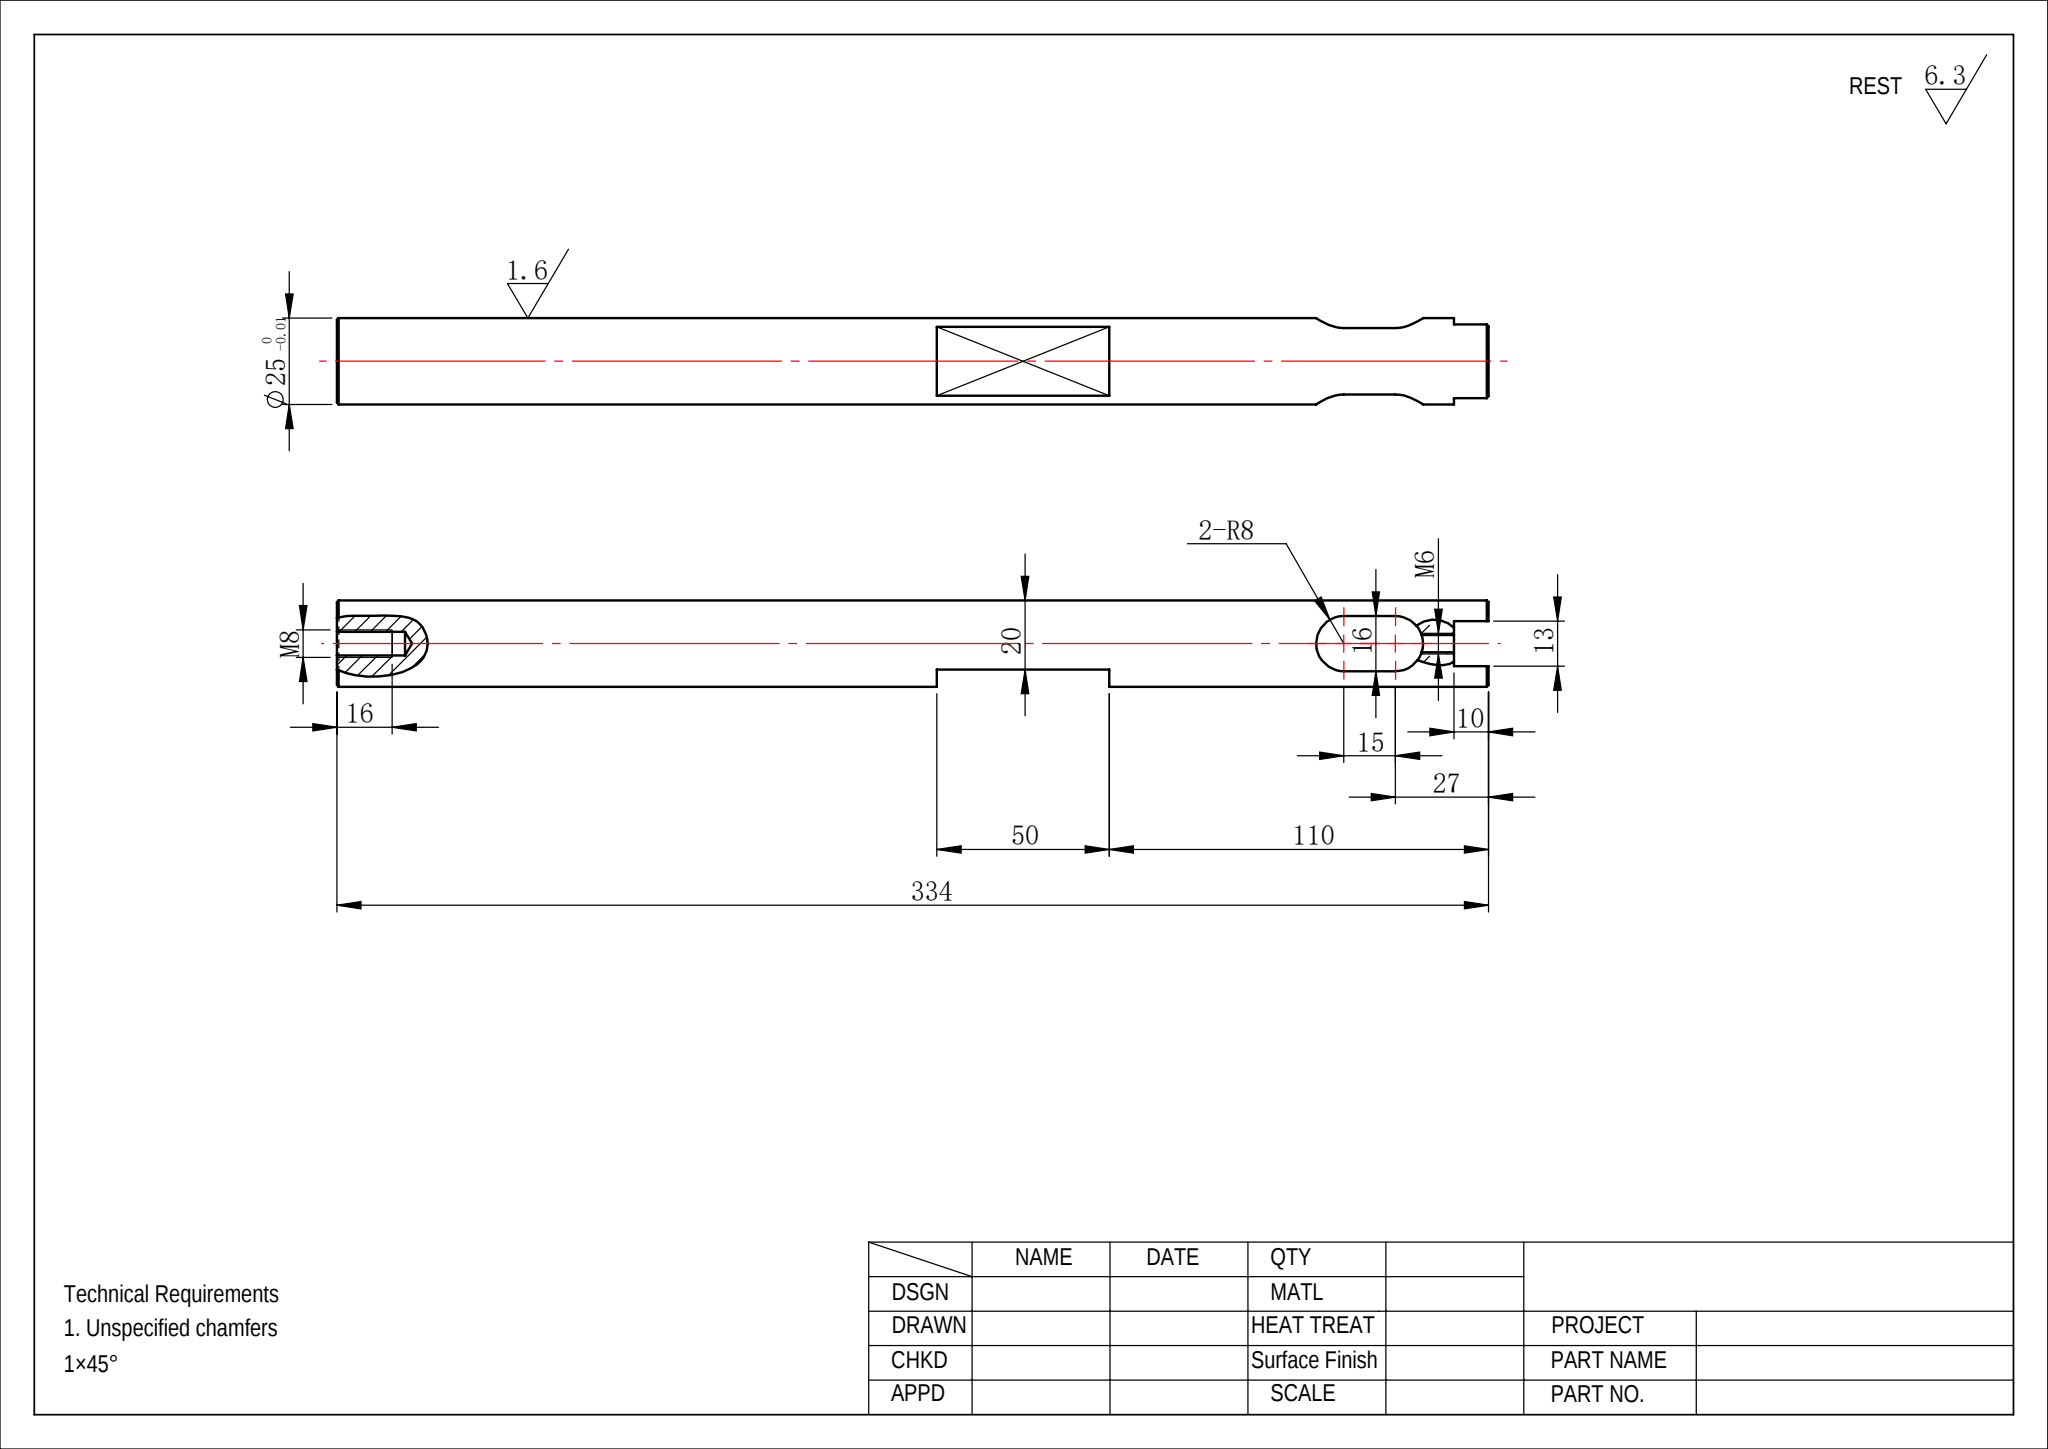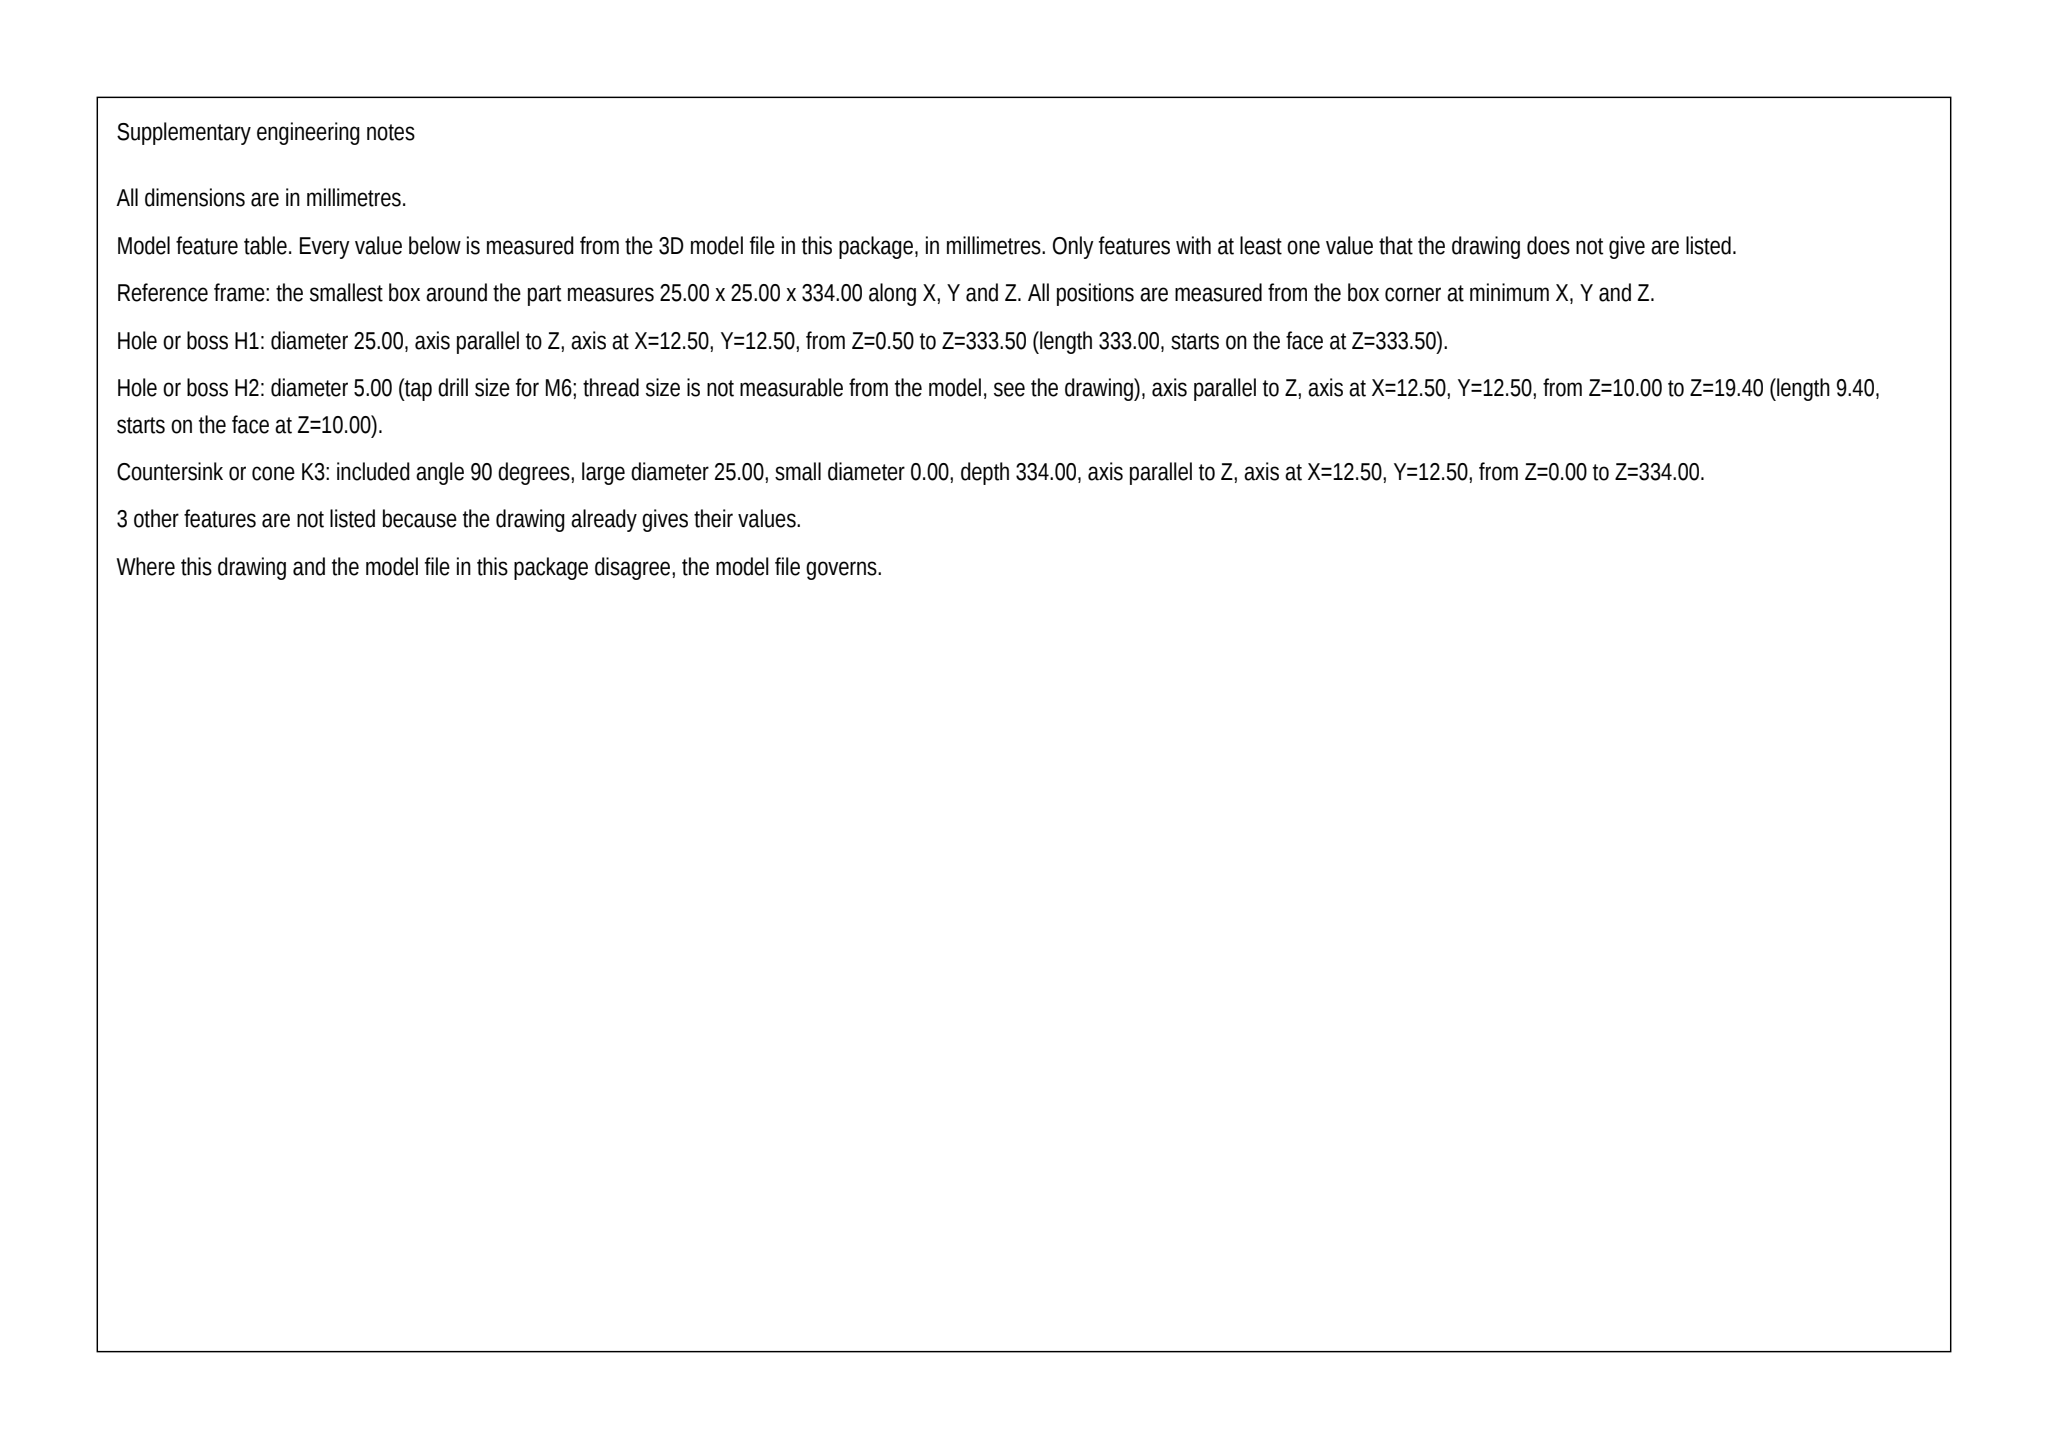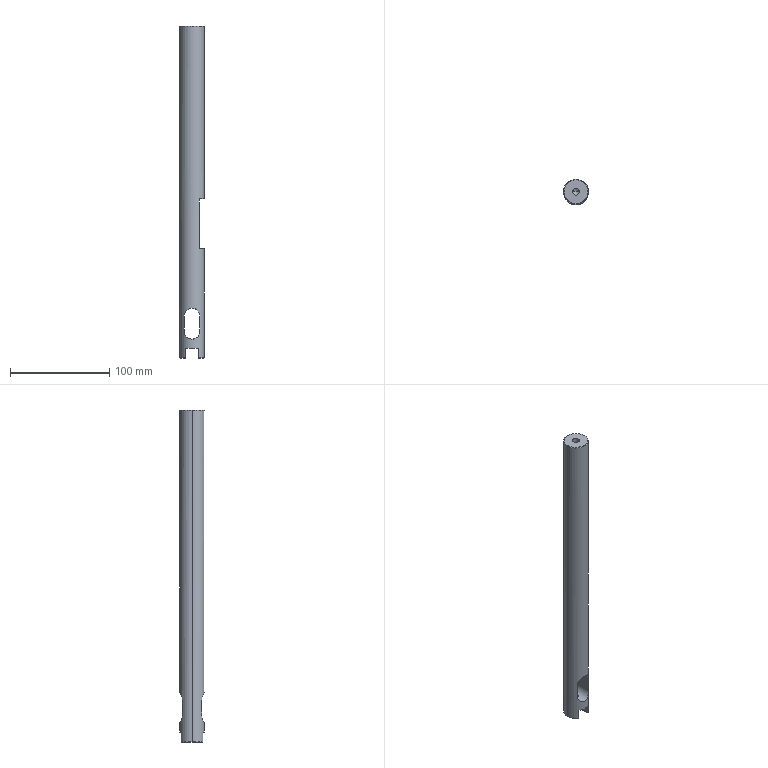Part | SolidWorks | mm | 1 solid | 27 faces | box 25 x 25 x 334 mm | volume 146109 mm3 | plane 11 | cylinder 9 | cone 7 | commonest cylinder face diameters 16 x3 5 x2 6.8 x2 25 x2
build123d program:
from build123d import *

# Parameters (mm, degrees)
SKETCH1_R             = 12.5
EXTRUDE1_DEPTH        = 334
SKETCH2_W             = 13
SKETCH2_H             = 26.185
CUT_EXTRUDE1_DEPTH    = 10
M8_TAPPED_HOLE1_D     = 6.8
M8_TAPPED_HOLE1_DEPTH = 19.75
M8_TAPPED_HOLE1_TIP   = 2.043
CUT_EXTRUDE3_DEPTH    = 25
SKETCH12_W            = 12.5
SKETCH12_H            = 10
SKETCH13_W            = 50
SKETCH13_H            = 120.795
CUT_EXTRUDE4_DEPTH    = 5
CHAMFER1_SIZE         = 0.5
M6_TAPPED_HOLE1_D     = 5
M6_TAPPED_HOLE1_DEPTH = 17
M6_TAPPED_HOLE1_TIP   = 1.502
SKETCH15_W            = 23.242
SKETCH15_H            = 67.222


with BuildPart() as part:
    # Sketch1 → Extrude1 (new body)
    with BuildSketch(Plane.XY):
        with Locations(Location((0, 0, 0), (0, 0, 180))):
            Circle(SKETCH1_R)
    extrude(amount=EXTRUDE1_DEPTH)

    # Sketch2 → Cut-Extrude1 (cut)
    with BuildSketch(Plane(origin=(0, 0, 0), x_dir=(-1, 0, 0), z_dir=(0, 0, -1))):
        with Locations((0, 0.2525)):
            Rectangle(SKETCH2_W, SKETCH2_H)
    extrude(amount=-CUT_EXTRUDE1_DEPTH, mode=Mode.SUBTRACT)

    # M8 Tapped Hole1
    with Locations(Plane.XY.offset(334)):
        with Locations((0, 0)):
            Hole(M8_TAPPED_HOLE1_D / 2, depth=M8_TAPPED_HOLE1_DEPTH)
            with Locations((0, 0, -(M8_TAPPED_HOLE1_DEPTH + M8_TAPPED_HOLE1_TIP / 2))):  # 118° drill point
                Cone(0, M8_TAPPED_HOLE1_D / 2, M8_TAPPED_HOLE1_TIP, mode=Mode.SUBTRACT)

    # Sketch7 → Cut-Extrude3 (cut, symmetric)
    with BuildSketch(Plane(origin=(0, 0, 0), x_dir=(1, 0, 0), z_dir=(0, 1, 0))):
        with BuildLine():
            Line((-8, -27), (-8, -42))
            ThreePointArc((-8, -42), (0, -50), (8, -42))
            Line((8, -42), (8, -27))
            ThreePointArc((8, -27), (0, -19), (-8, -27))
        make_face()
    extrude(amount=CUT_EXTRUDE3_DEPTH, both=True, mode=Mode.SUBTRACT)

    # Sketch12 → Revolve1 (revolve)
    with BuildSketch(Plane(origin=(0, 0, 0), x_dir=(1, 0, 0), z_dir=(0, 1, 0)), mode=Mode.PRIVATE) as revolve1_sk:
        with Locations((18.75, -175)):
            Rectangle(SKETCH12_W, SKETCH12_H)
    revolve(revolve1_sk.sketch.rotate(Axis((0, 0, 0), (0, 0, 1)), 121.332), axis=Axis((0, 0, 0), (0, 0, 1)))

    # Sketch13 → Cut-Extrude4 (cut)
    with BuildSketch(Plane(origin=(12.5, 0, 0), x_dir=(0, 0, -1), z_dir=(1, 0, 0))):
        with Locations((-135, 2.689)):
            Rectangle(SKETCH13_W, SKETCH13_H)
    extrude(amount=-CUT_EXTRUDE4_DEPTH, mode=Mode.SUBTRACT)

    # Chamfer1
    chamfer1_edges = [part.edges().sort_by_distance(p)[0] for p in [
        (12.5, 0, 334),
        (-10.897, -6.124, 0),
        (12.5, 0, 0),
    ]]
    chamfer(chamfer1_edges, length=CHAMFER1_SIZE)

    # M6 Tapped Hole1
    with Locations(Plane(origin=(0, 0, 10), x_dir=(-1, 0, 0), z_dir=(0, 0, -1))):
        with Locations((0, 0)):
            Hole(M6_TAPPED_HOLE1_D / 2, depth=M6_TAPPED_HOLE1_DEPTH)
            with Locations((0, 0, -(M6_TAPPED_HOLE1_DEPTH + M6_TAPPED_HOLE1_TIP / 2))):  # 118° drill point
                Cone(0, M6_TAPPED_HOLE1_D / 2, M6_TAPPED_HOLE1_TIP, mode=Mode.SUBTRACT)

    # Sketch15 → Cut-Revolve1 (revolve, cut)
    with BuildSketch(Plane(origin=(0, 0, 0), x_dir=(1, 0, 0), z_dir=(0, 1, 0)), mode=Mode.PRIVATE) as cut_revolve1_sk:
        with Locations((24.121, -174.248)):
            Rectangle(SKETCH15_W, SKETCH15_H)
    revolve(cut_revolve1_sk.sketch.rotate(Axis((0, 0, 0), (0, 0, 1)), 121.332), axis=Axis((0, 0, 0), (0, 0, 1)), mode=Mode.SUBTRACT)


solid = part.part